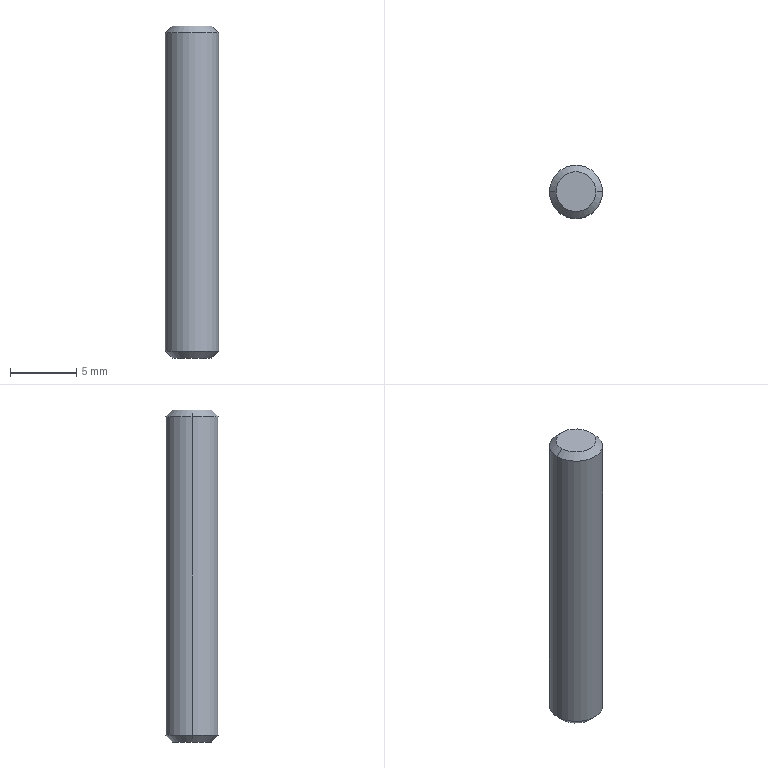Component | SolidWorks | 170423A4-DowelPin4x25-1 | 1 solid | 8 faces | box 4 x 4 x 25 mm | volume 311 mm3 | cone 4 | cylinder 2 | plane 2 | commonest cylinder face diameters 4 x2
build123d program:
from build123d import *

# Parameters (mm, degrees)
SKETCH1_R           = 2
BOSS_EXTRUDE1_DEPTH = 25
CHAMFER1_SIZE       = 0.5


with BuildPart() as part:
    # Sketch1 → Boss-Extrude1 (new body)
    with BuildSketch(Plane.XY):
        Circle(SKETCH1_R)
    extrude(amount=BOSS_EXTRUDE1_DEPTH)

    # Chamfer1
    chamfer1_edges = [part.edges().sort_by_distance(p)[0] for p in [
        (-2, 0, 0),
        (-2, 0, 25),
    ]]
    chamfer(chamfer1_edges, length=CHAMFER1_SIZE)


solid = part.part

# Placed as in the assembly
solid = solid.moved(Location((44.687, -75.611, -57.074), (0, 0, 0)))
STEP:
#1=COLOUR_RGB('',0.7922,0.8196,0.9333);
#2=FILL_AREA_STYLE_COLOUR('',#1);
#3=FILL_AREA_STYLE('',(#2));
#4=SURFACE_STYLE_FILL_AREA(#3);
#5=SURFACE_SIDE_STYLE('',(#4));
#6=SURFACE_STYLE_USAGE(.BOTH.,#5);
#7=PRESENTATION_STYLE_ASSIGNMENT((#6));
#8=CARTESIAN_POINT('',(1.818,-2.977,-1.263));
#9=VERTEX_POINT('',#8);
#10=CARTESIAN_POINT('',(1.7,-2.977,-1.263));
#11=VERTEX_POINT('',#10);
#12=CARTESIAN_POINT('',(1.759,-2.977,-1.263));
#13=DIRECTION('',(0.,0.,1.));
#14=DIRECTION('',(1.,0.,0.));
#15=AXIS2_PLACEMENT_3D('',#12,#13,#14);
#16=CIRCLE('',#15,0.05906);
#17=EDGE_CURVE('',#9,#11,#16,.T.);
#18=ORIENTED_EDGE('',*,*,#17,.F.);
#19=CARTESIAN_POINT('',(1.838,-2.977,-1.282));
#20=VERTEX_POINT('',#19);
#21=CARTESIAN_POINT('',(1.818,-2.977,-1.263));
#22=DIRECTION('',(0.7071,0.,-0.7071));
#23=VECTOR('',#22,39.37);
#24=LINE('',#21,#23);
#25=EDGE_CURVE('',#9,#20,#24,.T.);
#26=ORIENTED_EDGE('',*,*,#25,.T.);
#27=CARTESIAN_POINT('',(1.681,-2.977,-1.282));
#28=VERTEX_POINT('',#27);
#29=CARTESIAN_POINT('',(1.759,-2.977,-1.282));
#30=DIRECTION('',(0.,0.,-1.));
#31=DIRECTION('',(1.,0.,0.));
#32=AXIS2_PLACEMENT_3D('',#29,#30,#31);
#33=CIRCLE('',#32,0.07874);
#34=EDGE_CURVE('',#28,#20,#33,.T.);
#35=ORIENTED_EDGE('',*,*,#34,.F.);
#36=CARTESIAN_POINT('',(1.7,-2.977,-1.263));
#37=DIRECTION('',(-0.7071,0.,-0.7071));
#38=VECTOR('',#37,39.37);
#39=LINE('',#36,#38);
#40=EDGE_CURVE('',#11,#28,#39,.T.);
#41=ORIENTED_EDGE('',*,*,#40,.F.);
#42=EDGE_LOOP('',(#18,#26,#35,#41));
#43=FACE_OUTER_BOUND('',#42,.T.);
#44=CARTESIAN_POINT('',(1.759,-2.977,-1.263));
#45=DIRECTION('',(0.,0.,-1.));
#46=DIRECTION('',(-1.,0.,0.));
#47=AXIS2_PLACEMENT_3D('',#44,#45,#46);
#48=CONICAL_SURFACE('',#47,0.05906,0.7854);
#49=ADVANCED_FACE('',(#43),#48,.T.);
#50=CARTESIAN_POINT('',(1.7,-2.977,-2.247));
#51=VERTEX_POINT('',#50);
#52=CARTESIAN_POINT('',(1.818,-2.977,-2.247));
#53=VERTEX_POINT('',#52);
#54=CARTESIAN_POINT('',(1.759,-2.977,-2.247));
#55=DIRECTION('',(0.,0.,-1.));
#56=DIRECTION('',(1.,0.,0.));
#57=AXIS2_PLACEMENT_3D('',#54,#55,#56);
#58=CIRCLE('',#57,0.05906);
#59=EDGE_CURVE('',#51,#53,#58,.T.);
#60=ORIENTED_EDGE('',*,*,#59,.F.);
#61=CARTESIAN_POINT('',(1.681,-2.977,-2.227));
#62=VERTEX_POINT('',#61);
#63=CARTESIAN_POINT('',(1.681,-2.977,-2.227));
#64=DIRECTION('',(-0.7071,0.,0.7071));
#65=VECTOR('',#64,39.37);
#66=LINE('',#63,#65);
#67=EDGE_CURVE('',#51,#62,#66,.T.);
#68=ORIENTED_EDGE('',*,*,#67,.T.);
#69=CARTESIAN_POINT('',(1.838,-2.977,-2.227));
#70=VERTEX_POINT('',#69);
#71=CARTESIAN_POINT('',(1.759,-2.977,-2.227));
#72=DIRECTION('',(0.,0.,1.));
#73=DIRECTION('',(1.,0.,0.));
#74=AXIS2_PLACEMENT_3D('',#71,#72,#73);
#75=CIRCLE('',#74,0.07874);
#76=EDGE_CURVE('',#70,#62,#75,.T.);
#77=ORIENTED_EDGE('',*,*,#76,.F.);
#78=CARTESIAN_POINT('',(1.838,-2.977,-2.227));
#79=DIRECTION('',(0.7071,0.,0.7071));
#80=VECTOR('',#79,39.37);
#81=LINE('',#78,#80);
#82=EDGE_CURVE('',#53,#70,#81,.T.);
#83=ORIENTED_EDGE('',*,*,#82,.F.);
#84=EDGE_LOOP('',(#60,#68,#77,#83));
#85=FACE_OUTER_BOUND('',#84,.T.);
#86=CARTESIAN_POINT('',(1.759,-2.977,-2.227));
#87=DIRECTION('',(0.,0.,1.));
#88=DIRECTION('',(1.,0.,0.));
#89=AXIS2_PLACEMENT_3D('',#86,#87,#88);
#90=CONICAL_SURFACE('',#89,0.07874,0.7854);
#91=ADVANCED_FACE('',(#85),#90,.T.);
#92=ORIENTED_EDGE('',*,*,#34,.T.);
#93=CARTESIAN_POINT('',(1.838,-2.977,-1.263));
#94=DIRECTION('',(0.,0.,-1.));
#95=VECTOR('',#94,39.37);
#96=LINE('',#93,#95);
#97=EDGE_CURVE('',#20,#70,#96,.T.);
#98=ORIENTED_EDGE('',*,*,#97,.T.);
#99=ORIENTED_EDGE('',*,*,#76,.T.);
#100=CARTESIAN_POINT('',(1.681,-2.977,-1.263));
#101=DIRECTION('',(0.,0.,-1.));
#102=VECTOR('',#101,39.37);
#103=LINE('',#100,#102);
#104=EDGE_CURVE('',#28,#62,#103,.T.);
#105=ORIENTED_EDGE('',*,*,#104,.F.);
#106=EDGE_LOOP('',(#92,#98,#99,#105));
#107=FACE_OUTER_BOUND('',#106,.T.);
#108=CARTESIAN_POINT('',(1.759,-2.977,-1.263));
#109=DIRECTION('',(0.,0.,-1.));
#110=DIRECTION('',(-1.,0.,0.));
#111=AXIS2_PLACEMENT_3D('',#108,#109,#110);
#112=CYLINDRICAL_SURFACE('',#111,0.07874);
#113=ADVANCED_FACE('',(#107),#112,.T.);
#114=ORIENTED_EDGE('',*,*,#97,.F.);
#115=CARTESIAN_POINT('',(1.759,-2.977,-1.282));
#116=DIRECTION('',(0.,0.,-1.));
#117=DIRECTION('',(1.,0.,0.));
#118=AXIS2_PLACEMENT_3D('',#115,#116,#117);
#119=CIRCLE('',#118,0.07874);
#120=EDGE_CURVE('',#20,#28,#119,.T.);
#121=ORIENTED_EDGE('',*,*,#120,.T.);
#122=ORIENTED_EDGE('',*,*,#104,.T.);
#123=CARTESIAN_POINT('',(1.759,-2.977,-2.227));
#124=DIRECTION('',(0.,0.,1.));
#125=DIRECTION('',(1.,0.,0.));
#126=AXIS2_PLACEMENT_3D('',#123,#124,#125);
#127=CIRCLE('',#126,0.07874);
#128=EDGE_CURVE('',#62,#70,#127,.T.);
#129=ORIENTED_EDGE('',*,*,#128,.T.);
#130=EDGE_LOOP('',(#114,#121,#122,#129));
#131=FACE_OUTER_BOUND('',#130,.T.);
#132=CARTESIAN_POINT('',(1.759,-2.977,-1.263));
#133=DIRECTION('',(0.,0.,-1.));
#134=DIRECTION('',(-1.,0.,0.));
#135=AXIS2_PLACEMENT_3D('',#132,#133,#134);
#136=CYLINDRICAL_SURFACE('',#135,0.07874);
#137=ADVANCED_FACE('',(#131),#136,.T.);
#138=CARTESIAN_POINT('',(1.759,-2.977,-1.263));
#139=DIRECTION('',(0.,0.,1.));
#140=DIRECTION('',(1.,0.,0.));
#141=AXIS2_PLACEMENT_3D('',#138,#139,#140);
#142=CIRCLE('',#141,0.05906);
#143=EDGE_CURVE('',#11,#9,#142,.T.);
#144=ORIENTED_EDGE('',*,*,#143,.T.);
#145=ORIENTED_EDGE('',*,*,#17,.T.);
#146=EDGE_LOOP('',(#144,#145));
#147=FACE_OUTER_BOUND('',#146,.T.);
#148=CARTESIAN_POINT('',(1.759,-2.977,-1.263));
#149=DIRECTION('',(0.,0.,1.));
#150=DIRECTION('',(1.,0.,0.));
#151=AXIS2_PLACEMENT_3D('',#148,#149,#150);
#152=PLANE('',#151);
#153=ADVANCED_FACE('',(#147),#152,.T.);
#154=CARTESIAN_POINT('',(1.759,-2.977,-2.247));
#155=DIRECTION('',(0.,0.,-1.));
#156=DIRECTION('',(1.,0.,0.));
#157=AXIS2_PLACEMENT_3D('',#154,#155,#156);
#158=CIRCLE('',#157,0.05906);
#159=EDGE_CURVE('',#53,#51,#158,.T.);
#160=ORIENTED_EDGE('',*,*,#159,.T.);
#161=ORIENTED_EDGE('',*,*,#59,.T.);
#162=EDGE_LOOP('',(#160,#161));
#163=FACE_OUTER_BOUND('',#162,.T.);
#164=CARTESIAN_POINT('',(1.759,-2.977,-2.247));
#165=DIRECTION('',(0.,0.,1.));
#166=DIRECTION('',(1.,0.,0.));
#167=AXIS2_PLACEMENT_3D('',#164,#165,#166);
#168=PLANE('',#167);
#169=ADVANCED_FACE('',(#163),#168,.F.);
#170=ORIENTED_EDGE('',*,*,#67,.F.);
#171=ORIENTED_EDGE('',*,*,#159,.F.);
#172=ORIENTED_EDGE('',*,*,#82,.T.);
#173=ORIENTED_EDGE('',*,*,#128,.F.);
#174=EDGE_LOOP('',(#170,#171,#172,#173));
#175=FACE_OUTER_BOUND('',#174,.T.);
#176=CARTESIAN_POINT('',(1.759,-2.977,-2.227));
#177=DIRECTION('',(0.,0.,1.));
#178=DIRECTION('',(1.,0.,0.));
#179=AXIS2_PLACEMENT_3D('',#176,#177,#178);
#180=CONICAL_SURFACE('',#179,0.07874,0.7854);
#181=ADVANCED_FACE('',(#175),#180,.T.);
#182=ORIENTED_EDGE('',*,*,#25,.F.);
#183=ORIENTED_EDGE('',*,*,#143,.F.);
#184=ORIENTED_EDGE('',*,*,#40,.T.);
#185=ORIENTED_EDGE('',*,*,#120,.F.);
#186=EDGE_LOOP('',(#182,#183,#184,#185));
#187=FACE_OUTER_BOUND('',#186,.T.);
#188=CARTESIAN_POINT('',(1.759,-2.977,-1.263));
#189=DIRECTION('',(0.,0.,-1.));
#190=DIRECTION('',(-1.,0.,0.));
#191=AXIS2_PLACEMENT_3D('',#188,#189,#190);
#192=CONICAL_SURFACE('',#191,0.05906,0.7854);
#193=ADVANCED_FACE('',(#187),#192,.T.);
#194=CLOSED_SHELL('',(#49,#91,#113,#137,#153,#169,#181,#193));
#195=MANIFOLD_SOLID_BREP('',#194);
#196=STYLED_ITEM('',(#7),#195);
#197=(LENGTH_UNIT()NAMED_UNIT(*)SI_UNIT($,.METRE.));
#198=LENGTH_MEASURE_WITH_UNIT(LENGTH_MEASURE(0.0254),#197);
#199=DIMENSIONAL_EXPONENTS(1.,0.,0.,0.,0.,0.,0.);
#200=(CONVERSION_BASED_UNIT('',#198)LENGTH_UNIT()NAMED_UNIT(#199));
#201=UNCERTAINTY_MEASURE_WITH_UNIT(LENGTH_MEASURE(0.00001),#200,'','');
#202=(NAMED_UNIT(*)PLANE_ANGLE_UNIT()SI_UNIT($,.RADIAN.));
#203=(NAMED_UNIT(*)SI_UNIT($,.STERADIAN.)SOLID_ANGLE_UNIT());
#204=(GEOMETRIC_REPRESENTATION_CONTEXT(3)GLOBAL_UNCERTAINTY_ASSIGNED_CONTEXT((#201))GLOBAL_UNIT_ASSIGNED_CONTEXT((#200,#202,#203))REPRESENTATION_CONTEXT('',''));
#205=MECHANICAL_DESIGN_GEOMETRIC_PRESENTATION_REPRESENTATION('',(#196),#204);
#206=CARTESIAN_POINT('',(0.,0.,0.));
#207=DIRECTION('',(0.,0.,1.));
#208=DIRECTION('',(1.,0.,0.));
#209=AXIS2_PLACEMENT_3D('',#206,#207,#208);
#210=(LENGTH_UNIT()NAMED_UNIT(*)SI_UNIT($,.METRE.));
#211=LENGTH_MEASURE_WITH_UNIT(LENGTH_MEASURE(0.0254),#210);
#212=DIMENSIONAL_EXPONENTS(1.,0.,0.,0.,0.,0.,0.);
#213=(CONVERSION_BASED_UNIT('',#211)LENGTH_UNIT()NAMED_UNIT(#212));
#214=UNCERTAINTY_MEASURE_WITH_UNIT(LENGTH_MEASURE(0.00001),#213,'','');
#215=(NAMED_UNIT(*)PLANE_ANGLE_UNIT()SI_UNIT($,.RADIAN.));
#216=(NAMED_UNIT(*)SI_UNIT($,.STERADIAN.)SOLID_ANGLE_UNIT());
#217=(GEOMETRIC_REPRESENTATION_CONTEXT(3)GLOBAL_UNCERTAINTY_ASSIGNED_CONTEXT((#214))GLOBAL_UNIT_ASSIGNED_CONTEXT((#213,#215,#216))REPRESENTATION_CONTEXT('',''));
#218=ADVANCED_BREP_SHAPE_REPRESENTATION('',(#195,#209),#217);
#219=PRESENTATION_LAYER_ASSIGNMENT('','',(#196));